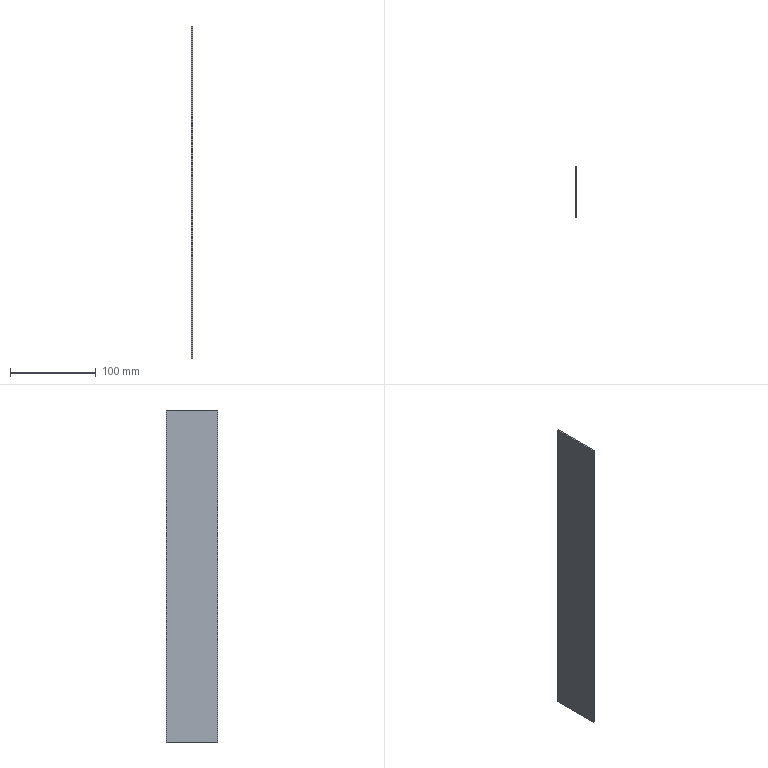Component | SolidWorks | SideBottomPlateBracket-1 | 1 solid | 6 faces | box 2 x 60 x 388 mm | volume 46560 mm3 | plane 6 | material Plain Carbon Steel
STEP:
#1=COLOUR_RGB('',0.7922,0.8196,0.9333);
#2=FILL_AREA_STYLE_COLOUR('',#1);
#3=FILL_AREA_STYLE('',(#2));
#4=SURFACE_STYLE_FILL_AREA(#3);
#5=SURFACE_SIDE_STYLE('',(#4));
#6=SURFACE_STYLE_USAGE(.BOTH.,#5);
#7=PRESENTATION_STYLE_ASSIGNMENT((#6));
#8=CARTESIAN_POINT('',(12.399,36.672,-3.564));
#9=VERTEX_POINT('',#8);
#10=CARTESIAN_POINT('',(12.399,39.034,-3.564));
#11=VERTEX_POINT('',#10);
#12=CARTESIAN_POINT('',(12.399,39.034,-3.564));
#13=DIRECTION('',(-0.,1.,0.));
#14=VECTOR('',#13,39.37);
#15=LINE('',#12,#14);
#16=EDGE_CURVE('',#9,#11,#15,.T.);
#17=ORIENTED_EDGE('',*,*,#16,.T.);
#18=CARTESIAN_POINT('',(12.399,39.034,11.712));
#19=VERTEX_POINT('',#18);
#20=CARTESIAN_POINT('',(12.399,39.034,11.712));
#21=DIRECTION('',(0.,0.,-1.));
#22=VECTOR('',#21,39.37);
#23=LINE('',#20,#22);
#24=EDGE_CURVE('',#19,#11,#23,.T.);
#25=ORIENTED_EDGE('',*,*,#24,.F.);
#26=CARTESIAN_POINT('',(12.399,36.672,11.712));
#27=VERTEX_POINT('',#26);
#28=CARTESIAN_POINT('',(12.399,39.034,11.712));
#29=DIRECTION('',(-0.,1.,0.));
#30=VECTOR('',#29,39.37);
#31=LINE('',#28,#30);
#32=EDGE_CURVE('',#27,#19,#31,.T.);
#33=ORIENTED_EDGE('',*,*,#32,.F.);
#34=CARTESIAN_POINT('',(12.399,36.672,11.712));
#35=DIRECTION('',(0.,0.,-1.));
#36=VECTOR('',#35,39.37);
#37=LINE('',#34,#36);
#38=EDGE_CURVE('',#27,#9,#37,.T.);
#39=ORIENTED_EDGE('',*,*,#38,.T.);
#40=EDGE_LOOP('',(#17,#25,#33,#39));
#41=FACE_OUTER_BOUND('',#40,.T.);
#42=CARTESIAN_POINT('',(12.399,39.034,11.712));
#43=DIRECTION('',(-1.,-0.,0.));
#44=DIRECTION('',(0.,-1.,0.));
#45=AXIS2_PLACEMENT_3D('',#42,#43,#44);
#46=PLANE('',#45);
#47=ADVANCED_FACE('',(#41),#46,.F.);
#48=CARTESIAN_POINT('',(12.321,39.034,-3.564));
#49=VERTEX_POINT('',#48);
#50=CARTESIAN_POINT('',(12.321,39.034,-3.564));
#51=DIRECTION('',(1.,-0.,0.));
#52=VECTOR('',#51,39.37);
#53=LINE('',#50,#52);
#54=EDGE_CURVE('',#49,#11,#53,.T.);
#55=ORIENTED_EDGE('',*,*,#54,.F.);
#56=CARTESIAN_POINT('',(12.321,39.034,11.712));
#57=VERTEX_POINT('',#56);
#58=CARTESIAN_POINT('',(12.321,39.034,11.712));
#59=DIRECTION('',(0.,0.,-1.));
#60=VECTOR('',#59,39.37);
#61=LINE('',#58,#60);
#62=EDGE_CURVE('',#57,#49,#61,.T.);
#63=ORIENTED_EDGE('',*,*,#62,.F.);
#64=CARTESIAN_POINT('',(12.321,39.034,11.712));
#65=DIRECTION('',(1.,-0.,0.));
#66=VECTOR('',#65,39.37);
#67=LINE('',#64,#66);
#68=EDGE_CURVE('',#57,#19,#67,.T.);
#69=ORIENTED_EDGE('',*,*,#68,.T.);
#70=ORIENTED_EDGE('',*,*,#24,.T.);
#71=EDGE_LOOP('',(#55,#63,#69,#70));
#72=FACE_OUTER_BOUND('',#71,.T.);
#73=CARTESIAN_POINT('',(12.321,39.034,11.712));
#74=DIRECTION('',(-0.,1.,0.));
#75=DIRECTION('',(0.,0.,1.));
#76=AXIS2_PLACEMENT_3D('',#73,#74,#75);
#77=PLANE('',#76);
#78=ADVANCED_FACE('',(#72),#77,.T.);
#79=CARTESIAN_POINT('',(12.321,36.672,-3.564));
#80=VERTEX_POINT('',#79);
#81=CARTESIAN_POINT('',(12.321,39.034,-3.564));
#82=DIRECTION('',(-0.,1.,0.));
#83=VECTOR('',#82,39.37);
#84=LINE('',#81,#83);
#85=EDGE_CURVE('',#80,#49,#84,.T.);
#86=ORIENTED_EDGE('',*,*,#85,.F.);
#87=CARTESIAN_POINT('',(12.321,36.672,11.712));
#88=VERTEX_POINT('',#87);
#89=CARTESIAN_POINT('',(12.321,36.672,11.712));
#90=DIRECTION('',(0.,0.,-1.));
#91=VECTOR('',#90,39.37);
#92=LINE('',#89,#91);
#93=EDGE_CURVE('',#88,#80,#92,.T.);
#94=ORIENTED_EDGE('',*,*,#93,.F.);
#95=CARTESIAN_POINT('',(12.321,39.034,11.712));
#96=DIRECTION('',(-0.,1.,0.));
#97=VECTOR('',#96,39.37);
#98=LINE('',#95,#97);
#99=EDGE_CURVE('',#88,#57,#98,.T.);
#100=ORIENTED_EDGE('',*,*,#99,.T.);
#101=ORIENTED_EDGE('',*,*,#62,.T.);
#102=EDGE_LOOP('',(#86,#94,#100,#101));
#103=FACE_OUTER_BOUND('',#102,.T.);
#104=CARTESIAN_POINT('',(12.321,39.034,11.712));
#105=DIRECTION('',(-1.,-0.,0.));
#106=DIRECTION('',(0.,-1.,0.));
#107=AXIS2_PLACEMENT_3D('',#104,#105,#106);
#108=PLANE('',#107);
#109=ADVANCED_FACE('',(#103),#108,.T.);
#110=CARTESIAN_POINT('',(12.399,36.672,-3.564));
#111=DIRECTION('',(-1.,0.,0.));
#112=VECTOR('',#111,39.37);
#113=LINE('',#110,#112);
#114=EDGE_CURVE('',#9,#80,#113,.T.);
#115=ORIENTED_EDGE('',*,*,#114,.F.);
#116=ORIENTED_EDGE('',*,*,#38,.F.);
#117=CARTESIAN_POINT('',(12.399,36.672,11.712));
#118=DIRECTION('',(-1.,0.,0.));
#119=VECTOR('',#118,39.37);
#120=LINE('',#117,#119);
#121=EDGE_CURVE('',#27,#88,#120,.T.);
#122=ORIENTED_EDGE('',*,*,#121,.T.);
#123=ORIENTED_EDGE('',*,*,#93,.T.);
#124=EDGE_LOOP('',(#115,#116,#122,#123));
#125=FACE_OUTER_BOUND('',#124,.T.);
#126=CARTESIAN_POINT('',(12.399,36.672,11.712));
#127=DIRECTION('',(0.,-1.,0.));
#128=DIRECTION('',(0.,0.,-1.));
#129=AXIS2_PLACEMENT_3D('',#126,#127,#128);
#130=PLANE('',#129);
#131=ADVANCED_FACE('',(#125),#130,.T.);
#132=ORIENTED_EDGE('',*,*,#32,.T.);
#133=ORIENTED_EDGE('',*,*,#68,.F.);
#134=ORIENTED_EDGE('',*,*,#99,.F.);
#135=ORIENTED_EDGE('',*,*,#121,.F.);
#136=EDGE_LOOP('',(#132,#133,#134,#135));
#137=FACE_OUTER_BOUND('',#136,.T.);
#138=CARTESIAN_POINT('',(15.629,37.599,11.712));
#139=DIRECTION('',(0.,0.,-1.));
#140=DIRECTION('',(-1.,0.,0.));
#141=AXIS2_PLACEMENT_3D('',#138,#139,#140);
#142=PLANE('',#141);
#143=ADVANCED_FACE('',(#137),#142,.F.);
#144=ORIENTED_EDGE('',*,*,#16,.F.);
#145=ORIENTED_EDGE('',*,*,#114,.T.);
#146=ORIENTED_EDGE('',*,*,#85,.T.);
#147=ORIENTED_EDGE('',*,*,#54,.T.);
#148=EDGE_LOOP('',(#144,#145,#146,#147));
#149=FACE_OUTER_BOUND('',#148,.T.);
#150=CARTESIAN_POINT('',(15.629,37.599,-3.564));
#151=DIRECTION('',(0.,0.,-1.));
#152=DIRECTION('',(-1.,0.,0.));
#153=AXIS2_PLACEMENT_3D('',#150,#151,#152);
#154=PLANE('',#153);
#155=ADVANCED_FACE('',(#149),#154,.T.);
#156=CLOSED_SHELL('',(#47,#78,#109,#131,#143,#155));
#157=MANIFOLD_SOLID_BREP('',#156);
#158=STYLED_ITEM('',(#7),#157);
#159=PRESENTATION_LAYER_ASSIGNMENT('','',(#158));
#160=(LENGTH_UNIT()NAMED_UNIT(*)SI_UNIT($,.METRE.));
#161=LENGTH_MEASURE_WITH_UNIT(LENGTH_MEASURE(0.0254),#160);
#162=DIMENSIONAL_EXPONENTS(1.,0.,0.,0.,0.,0.,0.);
#163=(CONVERSION_BASED_UNIT('',#161)LENGTH_UNIT()NAMED_UNIT(#162));
#164=UNCERTAINTY_MEASURE_WITH_UNIT(LENGTH_MEASURE(0.00001),#163,'','');
#165=(NAMED_UNIT(*)PLANE_ANGLE_UNIT()SI_UNIT($,.RADIAN.));
#166=(NAMED_UNIT(*)SI_UNIT($,.STERADIAN.)SOLID_ANGLE_UNIT());
#167=(GEOMETRIC_REPRESENTATION_CONTEXT(3)GLOBAL_UNCERTAINTY_ASSIGNED_CONTEXT((#164))GLOBAL_UNIT_ASSIGNED_CONTEXT((#163,#165,#166))REPRESENTATION_CONTEXT('',''));
#168=MECHANICAL_DESIGN_GEOMETRIC_PRESENTATION_REPRESENTATION('',(#158),#167);
#169=CARTESIAN_POINT('',(0.,0.,0.));
#170=DIRECTION('',(0.,0.,1.));
#171=DIRECTION('',(1.,0.,0.));
#172=AXIS2_PLACEMENT_3D('',#169,#170,#171);
#173=(LENGTH_UNIT()NAMED_UNIT(*)SI_UNIT($,.METRE.));
#174=LENGTH_MEASURE_WITH_UNIT(LENGTH_MEASURE(0.0254),#173);
#175=DIMENSIONAL_EXPONENTS(1.,0.,0.,0.,0.,0.,0.);
#176=(CONVERSION_BASED_UNIT('',#174)LENGTH_UNIT()NAMED_UNIT(#175));
#177=UNCERTAINTY_MEASURE_WITH_UNIT(LENGTH_MEASURE(0.00001),#176,'','');
#178=(NAMED_UNIT(*)PLANE_ANGLE_UNIT()SI_UNIT($,.RADIAN.));
#179=(NAMED_UNIT(*)SI_UNIT($,.STERADIAN.)SOLID_ANGLE_UNIT());
#180=(GEOMETRIC_REPRESENTATION_CONTEXT(3)GLOBAL_UNCERTAINTY_ASSIGNED_CONTEXT((#177))GLOBAL_UNIT_ASSIGNED_CONTEXT((#176,#178,#179))REPRESENTATION_CONTEXT('',''));
#181=ADVANCED_BREP_SHAPE_REPRESENTATION('',(#157,#172),#180);